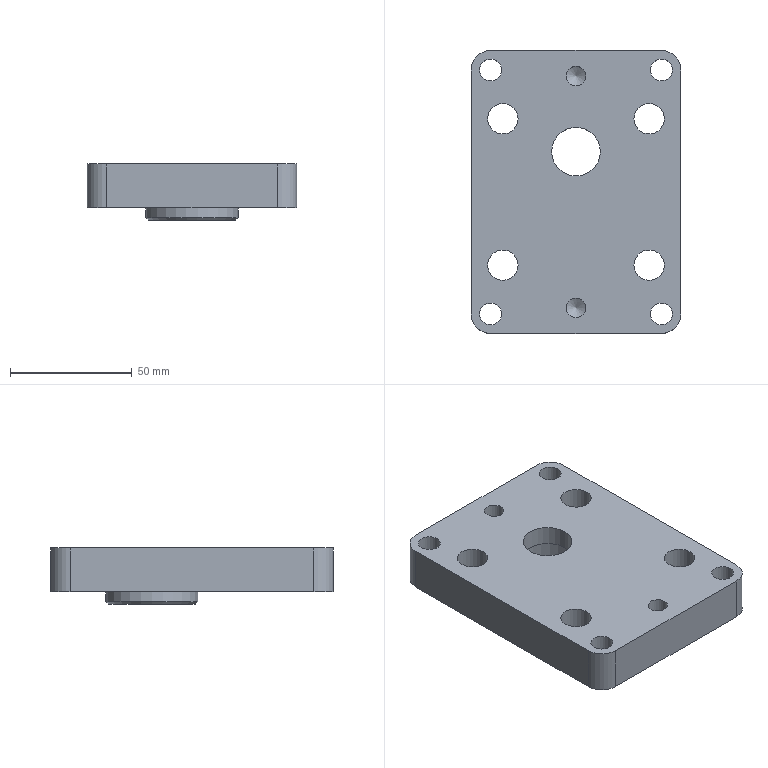Component | NX | 1 | 1 solid | 181 faces | volume 110268 mm3 | plane 145 | cylinder 32 | cone 4 | commonest cylinder face diameters 16 x8 18 x8 9 x4 12.5 x4 30 x2 8 x2 42 x1 38 x1